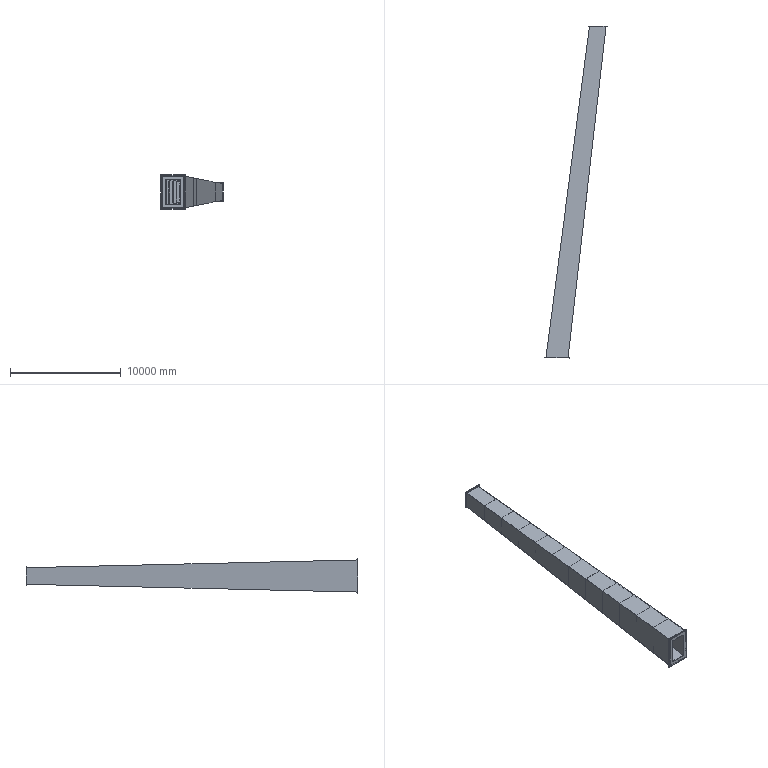Component | SolidWorks | RigidLeg-3 | 1 solid | 257 faces | volume 11320620667 mm3 | cylinder 142 | plane 89 | spline 26 | commonest cylinder face diameters 40 x140 200 x2